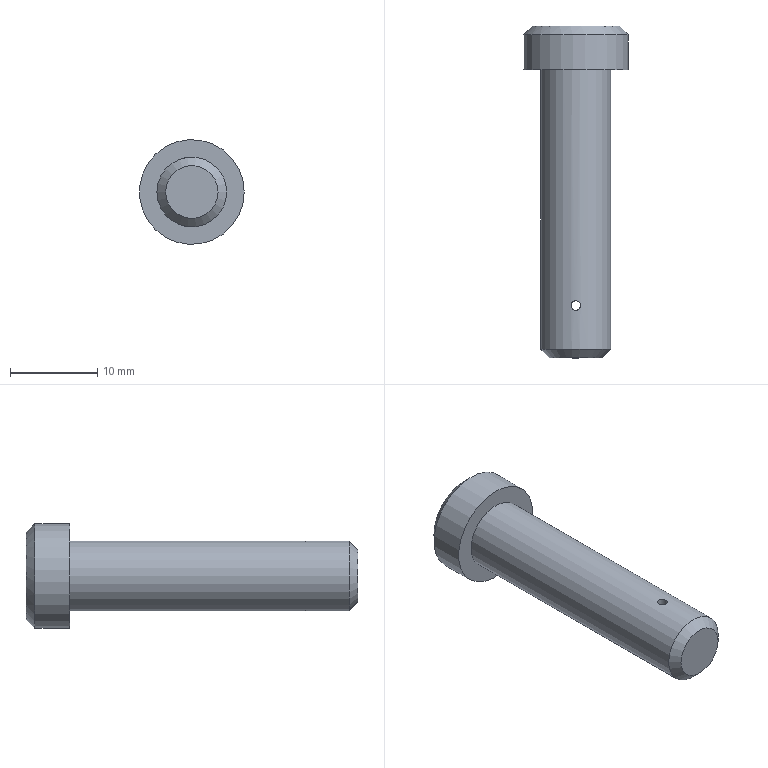Component | NX | SHAFT | 1 solid | 8 faces | box 12 x 38 x 12 mm | volume 2187 mm3 | cylinder 3 | plane 3 | cone 2 | commonest cylinder face diameters 8 x1 12 x1 1.1 x1
STEP:
#1=CARTESIAN_POINT('',(0.,0.,0.));
#2=DIRECTION('',(0.,0.,1.));
#3=DIRECTION('',(1.,0.,0.));
#4=AXIS2_PLACEMENT_3D('',#1,#2,#3);
#5=CARTESIAN_POINT('',(-77.,-19.5,-1.));
#6=VERTEX_POINT('',#5);
#7=CARTESIAN_POINT('',(-69.,-19.5,-1.));
#8=VERTEX_POINT('',#7);
#9=CARTESIAN_POINT('',(-73.,-19.5,-1.));
#10=DIRECTION('',(0.,1.,0.));
#11=DIRECTION('',(-1.,0.,0.));
#12=AXIS2_PLACEMENT_3D('',#9,#10,#11);
#13=CIRCLE('',#12,4.);
#14=CARTESIAN_POINT('',(-73.,-20.5,-1.));
#15=DIRECTION('',(0.,1.,0.));
#16=DIRECTION('',(1.,0.,0.));
#17=AXIS2_PLACEMENT_3D('',#14,#15,#16);
#18=CYLINDRICAL_SURFACE('',#17,4.);
#19=CARTESIAN_POINT('',(3.142,1.));
#20=DIRECTION('',(1.,0.));
#21=VECTOR('',#20,1.);
#22=LINE('',#19,#21);
#23=(GEOMETRIC_REPRESENTATION_CONTEXT(2)PARAMETRIC_REPRESENTATION_CONTEXT()REPRESENTATION_CONTEXT('',''));
#24=DEFINITIONAL_REPRESENTATION('',(#22),#23);
#25=PCURVE('',#18,#24);
#26=CARTESIAN_POINT('',(-73.,-19.5,-1.));
#27=DIRECTION('',(0.,1.,0.));
#28=DIRECTION('',(1.,0.,0.));
#29=AXIS2_PLACEMENT_3D('',#26,#27,#28);
#30=CONICAL_SURFACE('',#29,4.,0.7854);
#31=CARTESIAN_POINT('',(3.142,0.));
#32=DIRECTION('',(1.,0.));
#33=VECTOR('',#32,1.);
#34=LINE('',#31,#33);
#35=(GEOMETRIC_REPRESENTATION_CONTEXT(2)PARAMETRIC_REPRESENTATION_CONTEXT()REPRESENTATION_CONTEXT('',''));
#36=DEFINITIONAL_REPRESENTATION('',(#34),#35);
#37=PCURVE('',#30,#36);
#38=SURFACE_CURVE('',#13,(#25,#37),.PCURVE_S1.);
#39=EDGE_CURVE('',#6,#8,#38,.T.);
#40=ORIENTED_EDGE('',*,*,#39,.T.);
#41=CARTESIAN_POINT('',(-69.,12.5,-1.));
#42=VERTEX_POINT('',#41);
#43=CARTESIAN_POINT('',(-69.,-19.5,-1.));
#44=CARTESIAN_POINT('',(-69.,12.5,-1.));
#45=B_SPLINE_CURVE_WITH_KNOTS('',1,(#43,#44),.UNSPECIFIED.,.F.,.F.,(2,2),(1.,33.),.PIECEWISE_BEZIER_KNOTS.);
#46=CARTESIAN_POINT('',(6.283,0.));
#47=DIRECTION('',(0.,1.));
#48=VECTOR('',#47,1.);
#49=LINE('',#46,#48);
#50=(GEOMETRIC_REPRESENTATION_CONTEXT(2)PARAMETRIC_REPRESENTATION_CONTEXT()REPRESENTATION_CONTEXT('',''));
#51=DEFINITIONAL_REPRESENTATION('',(#49),#50);
#52=PCURVE('',#18,#51);
#53=CARTESIAN_POINT('',(0.,0.));
#54=DIRECTION('',(0.,1.));
#55=VECTOR('',#54,1.);
#56=LINE('',#53,#55);
#57=(GEOMETRIC_REPRESENTATION_CONTEXT(2)PARAMETRIC_REPRESENTATION_CONTEXT()REPRESENTATION_CONTEXT('',''));
#58=DEFINITIONAL_REPRESENTATION('',(#56),#57);
#59=PCURVE('',#18,#58);
#60=SEAM_CURVE('',#45,(#52,#59),.PCURVE_S1.);
#61=EDGE_CURVE('',#8,#42,#60,.T.);
#62=ORIENTED_EDGE('',*,*,#61,.T.);
#63=CARTESIAN_POINT('',(-73.,12.5,-1.));
#64=DIRECTION('',(0.,-1.,0.));
#65=DIRECTION('',(1.,0.,0.));
#66=AXIS2_PLACEMENT_3D('',#63,#64,#65);
#67=CIRCLE('',#66,4.);
#68=CARTESIAN_POINT('',(6.283,33.));
#69=DIRECTION('',(-1.,0.));
#70=VECTOR('',#69,1.);
#71=LINE('',#68,#70);
#72=(GEOMETRIC_REPRESENTATION_CONTEXT(2)PARAMETRIC_REPRESENTATION_CONTEXT()REPRESENTATION_CONTEXT('',''));
#73=DEFINITIONAL_REPRESENTATION('',(#71),#72);
#74=PCURVE('',#18,#73);
#75=CARTESIAN_POINT('',(-73.,12.5,-1.));
#76=DIRECTION('',(0.,-1.,0.));
#77=DIRECTION('',(-1.,0.,0.));
#78=AXIS2_PLACEMENT_3D('',#75,#76,#77);
#79=PLANE('',#78);
#80=CARTESIAN_POINT('',(0.,0.));
#81=DIRECTION('',(-1.,0.));
#82=AXIS2_PLACEMENT_2D('',#80,#81);
#83=CIRCLE('',#82,4.);
#84=(GEOMETRIC_REPRESENTATION_CONTEXT(2)PARAMETRIC_REPRESENTATION_CONTEXT()REPRESENTATION_CONTEXT('',''));
#85=DEFINITIONAL_REPRESENTATION('',(#83),#84);
#86=PCURVE('',#79,#85);
#87=SURFACE_CURVE('',#67,(#74,#86),.PCURVE_S1.);
#88=EDGE_CURVE('',#42,#42,#87,.T.);
#89=ORIENTED_EDGE('',*,*,#88,.T.);
#90=ORIENTED_EDGE('',*,*,#61,.F.);
#91=CARTESIAN_POINT('',(-73.,-19.5,-1.));
#92=DIRECTION('',(0.,1.,0.));
#93=DIRECTION('',(-1.,0.,0.));
#94=AXIS2_PLACEMENT_3D('',#91,#92,#93);
#95=CIRCLE('',#94,4.);
#96=CARTESIAN_POINT('',(-3.142,1.));
#97=DIRECTION('',(1.,0.));
#98=VECTOR('',#97,1.);
#99=LINE('',#96,#98);
#100=(GEOMETRIC_REPRESENTATION_CONTEXT(2)PARAMETRIC_REPRESENTATION_CONTEXT()REPRESENTATION_CONTEXT('',''));
#101=DEFINITIONAL_REPRESENTATION('',(#99),#100);
#102=PCURVE('',#18,#101);
#103=CARTESIAN_POINT('',(3.142,0.));
#104=DIRECTION('',(1.,0.));
#105=VECTOR('',#104,1.);
#106=LINE('',#103,#105);
#107=(GEOMETRIC_REPRESENTATION_CONTEXT(2)PARAMETRIC_REPRESENTATION_CONTEXT()REPRESENTATION_CONTEXT('',''));
#108=DEFINITIONAL_REPRESENTATION('',(#106),#107);
#109=PCURVE('',#30,#108);
#110=SURFACE_CURVE('',#95,(#102,#109),.PCURVE_S1.);
#111=EDGE_CURVE('',#8,#6,#110,.T.);
#112=ORIENTED_EDGE('',*,*,#111,.T.);
#113=EDGE_LOOP('',(#40,#62,#89,#90,#112));
#114=FACE_BOUND('',#113,.T.);
#115=CARTESIAN_POINT('',(-73.,-13.95,-5.));
#116=VERTEX_POINT('',#115);
#117=CARTESIAN_POINT('',(-73.,-13.95,-5.));
#118=CARTESIAN_POINT('',(-73.061,-13.95,-5.));
#119=CARTESIAN_POINT('',(-73.123,-13.961,-4.999));
#120=CARTESIAN_POINT('',(-73.181,-13.981,-4.996));
#121=CARTESIAN_POINT('',(-73.239,-14.001,-4.993));
#122=CARTESIAN_POINT('',(-73.294,-14.031,-4.989));
#123=CARTESIAN_POINT('',(-73.342,-14.069,-4.985));
#124=CARTESIAN_POINT('',(-73.39,-14.107,-4.981));
#125=CARTESIAN_POINT('',(-73.432,-14.154,-4.977));
#126=CARTESIAN_POINT('',(-73.465,-14.206,-4.973));
#127=CARTESIAN_POINT('',(-73.498,-14.258,-4.969));
#128=CARTESIAN_POINT('',(-73.522,-14.317,-4.966));
#129=CARTESIAN_POINT('',(-73.536,-14.377,-4.964));
#130=CARTESIAN_POINT('',(-73.55,-14.437,-4.962));
#131=CARTESIAN_POINT('',(-73.553,-14.5,-4.962));
#132=CARTESIAN_POINT('',(-73.547,-14.561,-4.962));
#133=CARTESIAN_POINT('',(-73.54,-14.622,-4.963));
#134=CARTESIAN_POINT('',(-73.523,-14.682,-4.966));
#135=CARTESIAN_POINT('',(-73.496,-14.737,-4.969));
#136=CARTESIAN_POINT('',(-73.47,-14.792,-4.972));
#137=CARTESIAN_POINT('',(-73.434,-14.844,-4.977));
#138=CARTESIAN_POINT('',(-73.391,-14.887,-4.981));
#139=CARTESIAN_POINT('',(-73.347,-14.931,-4.985));
#140=CARTESIAN_POINT('',(-73.296,-14.968,-4.989));
#141=CARTESIAN_POINT('',(-73.241,-14.995,-4.993));
#142=CARTESIAN_POINT('',(-73.185,-15.022,-4.996));
#143=CARTESIAN_POINT('',(-73.124,-15.039,-4.999));
#144=CARTESIAN_POINT('',(-73.063,-15.046,-5.));
#145=CARTESIAN_POINT('',(-73.002,-15.053,-5.));
#146=CARTESIAN_POINT('',(-72.939,-15.05,-5.));
#147=CARTESIAN_POINT('',(-72.879,-15.037,-4.998));
#148=CARTESIAN_POINT('',(-72.82,-15.023,-4.996));
#149=CARTESIAN_POINT('',(-72.762,-14.999,-4.993));
#150=CARTESIAN_POINT('',(-72.71,-14.967,-4.989));
#151=CARTESIAN_POINT('',(-72.658,-14.935,-4.986));
#152=CARTESIAN_POINT('',(-72.611,-14.893,-4.981));
#153=CARTESIAN_POINT('',(-72.572,-14.846,-4.977));
#154=CARTESIAN_POINT('',(-72.534,-14.798,-4.973));
#155=CARTESIAN_POINT('',(-72.502,-14.742,-4.969));
#156=CARTESIAN_POINT('',(-72.482,-14.684,-4.966));
#157=CARTESIAN_POINT('',(-72.461,-14.626,-4.964));
#158=CARTESIAN_POINT('',(-72.45,-14.564,-4.962));
#159=CARTESIAN_POINT('',(-72.45,-14.502,-4.962));
#160=CARTESIAN_POINT('',(-72.45,-14.441,-4.962));
#161=CARTESIAN_POINT('',(-72.46,-14.379,-4.963));
#162=CARTESIAN_POINT('',(-72.48,-14.321,-4.966));
#163=CARTESIAN_POINT('',(-72.5,-14.264,-4.969));
#164=CARTESIAN_POINT('',(-72.53,-14.209,-4.972));
#165=CARTESIAN_POINT('',(-72.567,-14.161,-4.977));
#166=CARTESIAN_POINT('',(-72.605,-14.112,-4.981));
#167=CARTESIAN_POINT('',(-72.652,-14.07,-4.985));
#168=CARTESIAN_POINT('',(-72.704,-14.037,-4.989));
#169=CARTESIAN_POINT('',(-72.756,-14.003,-4.993));
#170=CARTESIAN_POINT('',(-72.814,-13.979,-4.996));
#171=CARTESIAN_POINT('',(-72.874,-13.965,-4.998));
#172=CARTESIAN_POINT('',(-72.915,-13.955,-4.999));
#173=CARTESIAN_POINT('',(-72.958,-13.95,-5.));
#174=CARTESIAN_POINT('',(-73.,-13.95,-5.));
#175=B_SPLINE_CURVE_WITH_KNOTS('',3,(#117,#118,#119,#120,#121,#122,#123,#124,#125,#126,#127,#128,#129,#130,#131,#132,#133,#134,#135,#136,#137,#138,#139,#140,#141,#142,#143,#144,#145,#146,#147,#148,#149,#150,#151,#152,#153,#154,#155,#156,#157,#158,#159,#160,#161,#162,#163,#164,#165,#166,#167,#168,#169,#170,#171,#172,#173,#174),.UNSPECIFIED.,.T.,.F.,(1,3,3,3,3,3,3,3,3,3,3,3,3,3,3,3,3,3,3,3,3,1),(-0.03651,0.,0.05336,0.1067,0.1604,0.2142,0.2678,0.3209,0.3743,0.4281,0.4819,0.5353,0.5884,0.6419,0.6958,0.7495,0.8027,0.856,0.9096,0.9635,1.,1.053),.UNSPECIFIED.);
#176=CARTESIAN_POINT('',(1.571,6.55));
#177=CARTESIAN_POINT('',(1.574,6.55));
#178=CARTESIAN_POINT('',(1.581,6.549));
#179=CARTESIAN_POINT('',(1.59,6.545));
#180=CARTESIAN_POINT('',(1.6,6.538));
#181=CARTESIAN_POINT('',(1.61,6.528));
#182=CARTESIAN_POINT('',(1.619,6.516));
#183=CARTESIAN_POINT('',(1.628,6.501));
#184=CARTESIAN_POINT('',(1.637,6.483));
#185=CARTESIAN_POINT('',(1.645,6.463));
#186=CARTESIAN_POINT('',(1.653,6.441));
#187=CARTESIAN_POINT('',(1.661,6.416));
#188=CARTESIAN_POINT('',(1.668,6.389));
#189=CARTESIAN_POINT('',(1.675,6.361));
#190=CARTESIAN_POINT('',(1.681,6.33));
#191=CARTESIAN_POINT('',(1.687,6.298));
#192=CARTESIAN_POINT('',(1.692,6.264));
#193=CARTESIAN_POINT('',(1.696,6.229));
#194=CARTESIAN_POINT('',(1.7,6.193));
#195=CARTESIAN_POINT('',(1.703,6.155));
#196=CARTESIAN_POINT('',(1.706,6.117));
#197=CARTESIAN_POINT('',(1.707,6.079));
#198=CARTESIAN_POINT('',(1.708,6.039));
#199=CARTESIAN_POINT('',(1.709,6.));
#200=CARTESIAN_POINT('',(1.708,5.961));
#201=CARTESIAN_POINT('',(1.707,5.922));
#202=CARTESIAN_POINT('',(1.706,5.883));
#203=CARTESIAN_POINT('',(1.703,5.845));
#204=CARTESIAN_POINT('',(1.7,5.808));
#205=CARTESIAN_POINT('',(1.696,5.771));
#206=CARTESIAN_POINT('',(1.692,5.736));
#207=CARTESIAN_POINT('',(1.687,5.703));
#208=CARTESIAN_POINT('',(1.681,5.67));
#209=CARTESIAN_POINT('',(1.675,5.64));
#210=CARTESIAN_POINT('',(1.668,5.611));
#211=CARTESIAN_POINT('',(1.661,5.584));
#212=CARTESIAN_POINT('',(1.653,5.56));
#213=CARTESIAN_POINT('',(1.645,5.537));
#214=CARTESIAN_POINT('',(1.637,5.517));
#215=CARTESIAN_POINT('',(1.628,5.499));
#216=CARTESIAN_POINT('',(1.619,5.484));
#217=CARTESIAN_POINT('',(1.61,5.472));
#218=CARTESIAN_POINT('',(1.6,5.462));
#219=CARTESIAN_POINT('',(1.59,5.455));
#220=CARTESIAN_POINT('',(1.581,5.451));
#221=CARTESIAN_POINT('',(1.571,5.45));
#222=CARTESIAN_POINT('',(1.561,5.451));
#223=CARTESIAN_POINT('',(1.551,5.455));
#224=CARTESIAN_POINT('',(1.542,5.462));
#225=CARTESIAN_POINT('',(1.532,5.472));
#226=CARTESIAN_POINT('',(1.523,5.484));
#227=CARTESIAN_POINT('',(1.514,5.499));
#228=CARTESIAN_POINT('',(1.505,5.517));
#229=CARTESIAN_POINT('',(1.496,5.537));
#230=CARTESIAN_POINT('',(1.488,5.559));
#231=CARTESIAN_POINT('',(1.481,5.584));
#232=CARTESIAN_POINT('',(1.473,5.611));
#233=CARTESIAN_POINT('',(1.467,5.639));
#234=CARTESIAN_POINT('',(1.46,5.67));
#235=CARTESIAN_POINT('',(1.455,5.702));
#236=CARTESIAN_POINT('',(1.45,5.736));
#237=CARTESIAN_POINT('',(1.445,5.771));
#238=CARTESIAN_POINT('',(1.442,5.807));
#239=CARTESIAN_POINT('',(1.438,5.844));
#240=CARTESIAN_POINT('',(1.436,5.882));
#241=CARTESIAN_POINT('',(1.434,5.921));
#242=CARTESIAN_POINT('',(1.433,5.96));
#243=CARTESIAN_POINT('',(1.433,5.999));
#244=CARTESIAN_POINT('',(1.433,6.039));
#245=CARTESIAN_POINT('',(1.434,6.078));
#246=CARTESIAN_POINT('',(1.436,6.117));
#247=CARTESIAN_POINT('',(1.438,6.155));
#248=CARTESIAN_POINT('',(1.441,6.192));
#249=CARTESIAN_POINT('',(1.445,6.228));
#250=CARTESIAN_POINT('',(1.45,6.263));
#251=CARTESIAN_POINT('',(1.455,6.297));
#252=CARTESIAN_POINT('',(1.46,6.33));
#253=CARTESIAN_POINT('',(1.467,6.36));
#254=CARTESIAN_POINT('',(1.473,6.389));
#255=CARTESIAN_POINT('',(1.48,6.416));
#256=CARTESIAN_POINT('',(1.488,6.44));
#257=CARTESIAN_POINT('',(1.496,6.463));
#258=CARTESIAN_POINT('',(1.505,6.483));
#259=CARTESIAN_POINT('',(1.513,6.5));
#260=CARTESIAN_POINT('',(1.523,6.515));
#261=CARTESIAN_POINT('',(1.532,6.528));
#262=CARTESIAN_POINT('',(1.541,6.538));
#263=CARTESIAN_POINT('',(1.551,6.545));
#264=CARTESIAN_POINT('',(1.561,6.549));
#265=CARTESIAN_POINT('',(1.568,6.55));
#266=CARTESIAN_POINT('',(1.571,6.55));
#267=B_SPLINE_CURVE_WITH_KNOTS('',3,(#176,#177,#178,#179,#180,#181,#182,#183,#184,#185,#186,#187,#188,#189,#190,#191,#192,#193,#194,#195,#196,#197,#198,#199,#200,#201,#202,#203,#204,#205,#206,#207,#208,#209,#210,#211,#212,#213,#214,#215,#216,#217,#218,#219,#220,#221,#222,#223,#224,#225,#226,#227,#228,#229,#230,#231,#232,#233,#234,#235,#236,#237,#238,#239,#240,#241,#242,#243,#244,#245,#246,#247,#248,#249,#250,#251,#252,#253,#254,#255,#256,#257,#258,#259,#260,#261,#262,#263,#264,#265,#266),.UNSPECIFIED.,.T.,.F.,(4,1,1,1,1,1,1,1,1,1,1,1,1,1,1,1,1,1,1,1,1,1,1,1,1,1,1,1,1,1,1,1,1,1,1,1,1,1,1,1,1,1,1,1,1,1,1,1,1,1,1,1,1,1,1,1,1,1,1,1,1,1,1,1,1,1,1,1,1,1,1,1,1,1,1,1,1,1,1,1,1,1,1,1,1,1,1,1,4),(0.,0.01136,0.02273,0.03409,0.04545,0.05682,0.06818,0.07955,0.09091,0.1023,0.1136,0.125,0.1364,0.1477,0.1591,0.1705,0.1818,0.1932,0.2045,0.2159,0.2273,0.2386,0.25,0.2614,0.2727,0.2841,0.2955,0.3068,0.3182,0.3295,0.3409,0.3523,0.3636,0.375,0.3864,0.3977,0.4091,0.4205,0.4318,0.4432,0.4545,0.4659,0.4773,0.4886,0.5,0.5114,0.5227,0.5341,0.5455,0.5568,0.5682,0.5795,0.5909,0.6023,0.6136,0.625,0.6364,0.6477,0.6591,0.6705,0.6818,0.6932,0.7045,0.7159,0.7273,0.7386,0.75,0.7614,0.7727,0.7841,0.7955,0.8068,0.8182,0.8295,0.8409,0.8523,0.8636,0.875,0.8864,0.8977,0.9091,0.9205,0.9318,0.9432,0.9545,0.9659,0.9773,0.9886,1.),.QUASI_UNIFORM_KNOTS.);
#268=(GEOMETRIC_REPRESENTATION_CONTEXT(2)PARAMETRIC_REPRESENTATION_CONTEXT()REPRESENTATION_CONTEXT('',''));
#269=DEFINITIONAL_REPRESENTATION('',(#267),#268);
#270=PCURVE('',#18,#269);
#271=CARTESIAN_POINT('',(-73.,-14.5,29.));
#272=DIRECTION('',(0.,0.,-1.));
#273=DIRECTION('',(0.,1.,0.));
#274=AXIS2_PLACEMENT_3D('',#271,#272,#273);
#275=CYLINDRICAL_SURFACE('',#274,0.55);
#276=CARTESIAN_POINT('',(6.283,34.));
#277=CARTESIAN_POINT('',(0.,34.));
#278=B_SPLINE_CURVE_WITH_KNOTS('',1,(#276,#277),.UNSPECIFIED.,.F.,.F.,(2,2),(0.,1.),.PIECEWISE_BEZIER_KNOTS.);
#279=(GEOMETRIC_REPRESENTATION_CONTEXT(2)PARAMETRIC_REPRESENTATION_CONTEXT()REPRESENTATION_CONTEXT('',''));
#280=DEFINITIONAL_REPRESENTATION('',(#278),#279);
#281=PCURVE('',#275,#280);
#282=SURFACE_CURVE('',#175,(#270,#281),.PCURVE_S1.);
#283=EDGE_CURVE('',#116,#116,#282,.T.);
#284=ORIENTED_EDGE('',*,*,#283,.T.);
#285=EDGE_LOOP('',(#284));
#286=FACE_BOUND('',#285,.T.);
#287=CARTESIAN_POINT('',(-73.,-13.95,3.));
#288=VERTEX_POINT('',#287);
#289=CARTESIAN_POINT('',(-73.,-13.95,3.));
#290=CARTESIAN_POINT('',(-72.939,-13.95,3.));
#291=CARTESIAN_POINT('',(-72.877,-13.961,2.999));
#292=CARTESIAN_POINT('',(-72.819,-13.981,2.996));
#293=CARTESIAN_POINT('',(-72.761,-14.001,2.993));
#294=CARTESIAN_POINT('',(-72.706,-14.031,2.989));
#295=CARTESIAN_POINT('',(-72.658,-14.069,2.985));
#296=CARTESIAN_POINT('',(-72.61,-14.107,2.981));
#297=CARTESIAN_POINT('',(-72.568,-14.154,2.977));
#298=CARTESIAN_POINT('',(-72.535,-14.206,2.973));
#299=CARTESIAN_POINT('',(-72.502,-14.258,2.969));
#300=CARTESIAN_POINT('',(-72.478,-14.317,2.966));
#301=CARTESIAN_POINT('',(-72.464,-14.377,2.964));
#302=CARTESIAN_POINT('',(-72.45,-14.437,2.962));
#303=CARTESIAN_POINT('',(-72.447,-14.5,2.962));
#304=CARTESIAN_POINT('',(-72.453,-14.561,2.962));
#305=CARTESIAN_POINT('',(-72.46,-14.622,2.963));
#306=CARTESIAN_POINT('',(-72.477,-14.682,2.966));
#307=CARTESIAN_POINT('',(-72.504,-14.737,2.969));
#308=CARTESIAN_POINT('',(-72.53,-14.792,2.972));
#309=CARTESIAN_POINT('',(-72.566,-14.844,2.977));
#310=CARTESIAN_POINT('',(-72.609,-14.887,2.981));
#311=CARTESIAN_POINT('',(-72.653,-14.931,2.985));
#312=CARTESIAN_POINT('',(-72.704,-14.968,2.989));
#313=CARTESIAN_POINT('',(-72.759,-14.995,2.993));
#314=CARTESIAN_POINT('',(-72.815,-15.022,2.996));
#315=CARTESIAN_POINT('',(-72.876,-15.039,2.999));
#316=CARTESIAN_POINT('',(-72.937,-15.046,3.));
#317=CARTESIAN_POINT('',(-72.998,-15.053,3.));
#318=CARTESIAN_POINT('',(-73.061,-15.05,3.));
#319=CARTESIAN_POINT('',(-73.121,-15.037,2.998));
#320=CARTESIAN_POINT('',(-73.18,-15.023,2.996));
#321=CARTESIAN_POINT('',(-73.238,-14.999,2.993));
#322=CARTESIAN_POINT('',(-73.29,-14.967,2.989));
#323=CARTESIAN_POINT('',(-73.342,-14.935,2.986));
#324=CARTESIAN_POINT('',(-73.389,-14.893,2.981));
#325=CARTESIAN_POINT('',(-73.428,-14.846,2.977));
#326=CARTESIAN_POINT('',(-73.466,-14.798,2.973));
#327=CARTESIAN_POINT('',(-73.498,-14.742,2.969));
#328=CARTESIAN_POINT('',(-73.518,-14.684,2.966));
#329=CARTESIAN_POINT('',(-73.539,-14.626,2.964));
#330=CARTESIAN_POINT('',(-73.55,-14.564,2.962));
#331=CARTESIAN_POINT('',(-73.55,-14.502,2.962));
#332=CARTESIAN_POINT('',(-73.55,-14.441,2.962));
#333=CARTESIAN_POINT('',(-73.54,-14.379,2.963));
#334=CARTESIAN_POINT('',(-73.52,-14.321,2.966));
#335=CARTESIAN_POINT('',(-73.5,-14.264,2.969));
#336=CARTESIAN_POINT('',(-73.47,-14.209,2.972));
#337=CARTESIAN_POINT('',(-73.433,-14.161,2.977));
#338=CARTESIAN_POINT('',(-73.395,-14.112,2.981));
#339=CARTESIAN_POINT('',(-73.348,-14.07,2.985));
#340=CARTESIAN_POINT('',(-73.296,-14.037,2.989));
#341=CARTESIAN_POINT('',(-73.244,-14.003,2.993));
#342=CARTESIAN_POINT('',(-73.186,-13.979,2.996));
#343=CARTESIAN_POINT('',(-73.126,-13.965,2.998));
#344=CARTESIAN_POINT('',(-73.085,-13.955,2.999));
#345=CARTESIAN_POINT('',(-73.042,-13.95,3.));
#346=CARTESIAN_POINT('',(-73.,-13.95,3.));
#347=B_SPLINE_CURVE_WITH_KNOTS('',3,(#289,#290,#291,#292,#293,#294,#295,#296,#297,#298,#299,#300,#301,#302,#303,#304,#305,#306,#307,#308,#309,#310,#311,#312,#313,#314,#315,#316,#317,#318,#319,#320,#321,#322,#323,#324,#325,#326,#327,#328,#329,#330,#331,#332,#333,#334,#335,#336,#337,#338,#339,#340,#341,#342,#343,#344,#345,#346),.UNSPECIFIED.,.T.,.F.,(1,3,3,3,3,3,3,3,3,3,3,3,3,3,3,3,3,3,3,3,3,1),(-0.03651,0.,0.05336,0.1067,0.1604,0.2142,0.2678,0.3209,0.3743,0.4281,0.4819,0.5353,0.5884,0.6419,0.6958,0.7495,0.8027,0.856,0.9096,0.9635,1.,1.053),.UNSPECIFIED.);
#348=CARTESIAN_POINT('',(4.712,6.55));
#349=CARTESIAN_POINT('',(4.716,6.55));
#350=CARTESIAN_POINT('',(4.722,6.549));
#351=CARTESIAN_POINT('',(4.732,6.545));
#352=CARTESIAN_POINT('',(4.742,6.538));
#353=CARTESIAN_POINT('',(4.751,6.528));
#354=CARTESIAN_POINT('',(4.761,6.516));
#355=CARTESIAN_POINT('',(4.77,6.501));
#356=CARTESIAN_POINT('',(4.778,6.483));
#357=CARTESIAN_POINT('',(4.787,6.463));
#358=CARTESIAN_POINT('',(4.795,6.441));
#359=CARTESIAN_POINT('',(4.803,6.416));
#360=CARTESIAN_POINT('',(4.81,6.389));
#361=CARTESIAN_POINT('',(4.817,6.361));
#362=CARTESIAN_POINT('',(4.823,6.33));
#363=CARTESIAN_POINT('',(4.828,6.298));
#364=CARTESIAN_POINT('',(4.833,6.264));
#365=CARTESIAN_POINT('',(4.838,6.229));
#366=CARTESIAN_POINT('',(4.842,6.193));
#367=CARTESIAN_POINT('',(4.845,6.155));
#368=CARTESIAN_POINT('',(4.847,6.117));
#369=CARTESIAN_POINT('',(4.849,6.079));
#370=CARTESIAN_POINT('',(4.85,6.039));
#371=CARTESIAN_POINT('',(4.85,6.));
#372=CARTESIAN_POINT('',(4.85,5.961));
#373=CARTESIAN_POINT('',(4.849,5.922));
#374=CARTESIAN_POINT('',(4.847,5.883));
#375=CARTESIAN_POINT('',(4.845,5.845));
#376=CARTESIAN_POINT('',(4.842,5.808));
#377=CARTESIAN_POINT('',(4.838,5.771));
#378=CARTESIAN_POINT('',(4.833,5.736));
#379=CARTESIAN_POINT('',(4.828,5.703));
#380=CARTESIAN_POINT('',(4.823,5.67));
#381=CARTESIAN_POINT('',(4.817,5.64));
#382=CARTESIAN_POINT('',(4.81,5.611));
#383=CARTESIAN_POINT('',(4.803,5.584));
#384=CARTESIAN_POINT('',(4.795,5.56));
#385=CARTESIAN_POINT('',(4.787,5.537));
#386=CARTESIAN_POINT('',(4.778,5.517));
#387=CARTESIAN_POINT('',(4.77,5.499));
#388=CARTESIAN_POINT('',(4.761,5.484));
#389=CARTESIAN_POINT('',(4.751,5.472));
#390=CARTESIAN_POINT('',(4.742,5.462));
#391=CARTESIAN_POINT('',(4.732,5.455));
#392=CARTESIAN_POINT('',(4.722,5.451));
#393=CARTESIAN_POINT('',(4.712,5.45));
#394=CARTESIAN_POINT('',(4.703,5.451));
#395=CARTESIAN_POINT('',(4.693,5.455));
#396=CARTESIAN_POINT('',(4.683,5.462));
#397=CARTESIAN_POINT('',(4.674,5.472));
#398=CARTESIAN_POINT('',(4.664,5.484));
#399=CARTESIAN_POINT('',(4.655,5.499));
#400=CARTESIAN_POINT('',(4.646,5.517));
#401=CARTESIAN_POINT('',(4.638,5.537));
#402=CARTESIAN_POINT('',(4.63,5.559));
#403=CARTESIAN_POINT('',(4.622,5.584));
#404=CARTESIAN_POINT('',(4.615,5.611));
#405=CARTESIAN_POINT('',(4.608,5.639));
#406=CARTESIAN_POINT('',(4.602,5.67));
#407=CARTESIAN_POINT('',(4.596,5.702));
#408=CARTESIAN_POINT('',(4.591,5.736));
#409=CARTESIAN_POINT('',(4.587,5.771));
#410=CARTESIAN_POINT('',(4.583,5.807));
#411=CARTESIAN_POINT('',(4.58,5.844));
#412=CARTESIAN_POINT('',(4.578,5.882));
#413=CARTESIAN_POINT('',(4.576,5.921));
#414=CARTESIAN_POINT('',(4.575,5.96));
#415=CARTESIAN_POINT('',(4.574,5.999));
#416=CARTESIAN_POINT('',(4.575,6.039));
#417=CARTESIAN_POINT('',(4.576,6.078));
#418=CARTESIAN_POINT('',(4.578,6.117));
#419=CARTESIAN_POINT('',(4.58,6.155));
#420=CARTESIAN_POINT('',(4.583,6.192));
#421=CARTESIAN_POINT('',(4.587,6.228));
#422=CARTESIAN_POINT('',(4.591,6.263));
#423=CARTESIAN_POINT('',(4.596,6.297));
#424=CARTESIAN_POINT('',(4.602,6.33));
#425=CARTESIAN_POINT('',(4.608,6.36));
#426=CARTESIAN_POINT('',(4.615,6.389));
#427=CARTESIAN_POINT('',(4.622,6.416));
#428=CARTESIAN_POINT('',(4.63,6.44));
#429=CARTESIAN_POINT('',(4.638,6.463));
#430=CARTESIAN_POINT('',(4.646,6.483));
#431=CARTESIAN_POINT('',(4.655,6.5));
#432=CARTESIAN_POINT('',(4.664,6.515));
#433=CARTESIAN_POINT('',(4.673,6.528));
#434=CARTESIAN_POINT('',(4.683,6.538));
#435=CARTESIAN_POINT('',(4.693,6.545));
#436=CARTESIAN_POINT('',(4.703,6.549));
#437=CARTESIAN_POINT('',(4.709,6.55));
#438=CARTESIAN_POINT('',(4.712,6.55));
#439=B_SPLINE_CURVE_WITH_KNOTS('',3,(#348,#349,#350,#351,#352,#353,#354,#355,#356,#357,#358,#359,#360,#361,#362,#363,#364,#365,#366,#367,#368,#369,#370,#371,#372,#373,#374,#375,#376,#377,#378,#379,#380,#381,#382,#383,#384,#385,#386,#387,#388,#389,#390,#391,#392,#393,#394,#395,#396,#397,#398,#399,#400,#401,#402,#403,#404,#405,#406,#407,#408,#409,#410,#411,#412,#413,#414,#415,#416,#417,#418,#419,#420,#421,#422,#423,#424,#425,#426,#427,#428,#429,#430,#431,#432,#433,#434,#435,#436,#437,#438),.UNSPECIFIED.,.T.,.F.,(4,1,1,1,1,1,1,1,1,1,1,1,1,1,1,1,1,1,1,1,1,1,1,1,1,1,1,1,1,1,1,1,1,1,1,1,1,1,1,1,1,1,1,1,1,1,1,1,1,1,1,1,1,1,1,1,1,1,1,1,1,1,1,1,1,1,1,1,1,1,1,1,1,1,1,1,1,1,1,1,1,1,1,1,1,1,1,1,4),(0.,0.01136,0.02273,0.03409,0.04545,0.05682,0.06818,0.07955,0.09091,0.1023,0.1136,0.125,0.1364,0.1477,0.1591,0.1705,0.1818,0.1932,0.2045,0.2159,0.2273,0.2386,0.25,0.2614,0.2727,0.2841,0.2955,0.3068,0.3182,0.3295,0.3409,0.3523,0.3636,0.375,0.3864,0.3977,0.4091,0.4205,0.4318,0.4432,0.4545,0.4659,0.4773,0.4886,0.5,0.5114,0.5227,0.5341,0.5455,0.5568,0.5682,0.5795,0.5909,0.6023,0.6136,0.625,0.6364,0.6477,0.6591,0.6705,0.6818,0.6932,0.7045,0.7159,0.7273,0.7386,0.75,0.7614,0.7727,0.7841,0.7955,0.8068,0.8182,0.8295,0.8409,0.8523,0.8636,0.875,0.8864,0.8977,0.9091,0.9205,0.9318,0.9432,0.9545,0.9659,0.9773,0.9886,1.),.QUASI_UNIFORM_KNOTS.);
#440=(GEOMETRIC_REPRESENTATION_CONTEXT(2)PARAMETRIC_REPRESENTATION_CONTEXT()REPRESENTATION_CONTEXT('',''));
#441=DEFINITIONAL_REPRESENTATION('',(#439),#440);
#442=PCURVE('',#18,#441);
#443=CARTESIAN_POINT('',(0.,26.));
#444=CARTESIAN_POINT('',(6.283,26.));
#445=B_SPLINE_CURVE_WITH_KNOTS('',1,(#443,#444),.UNSPECIFIED.,.F.,.F.,(2,2),(0.,1.),.PIECEWISE_BEZIER_KNOTS.);
#446=(GEOMETRIC_REPRESENTATION_CONTEXT(2)PARAMETRIC_REPRESENTATION_CONTEXT()REPRESENTATION_CONTEXT('',''));
#447=DEFINITIONAL_REPRESENTATION('',(#445),#446);
#448=PCURVE('',#275,#447);
#449=SURFACE_CURVE('',#347,(#442,#448),.PCURVE_S1.);
#450=EDGE_CURVE('',#288,#288,#449,.T.);
#451=ORIENTED_EDGE('',*,*,#450,.T.);
#452=EDGE_LOOP('',(#451));
#453=FACE_BOUND('',#452,.T.);
#454=ADVANCED_FACE('',(#114,#286,#453),#18,.T.);
#455=CARTESIAN_POINT('',(-76.,-20.5,-1.));
#456=VERTEX_POINT('',#455);
#457=CARTESIAN_POINT('',(-73.,-20.5,-1.));
#458=DIRECTION('',(0.,-1.,0.));
#459=DIRECTION('',(-1.,0.,0.));
#460=AXIS2_PLACEMENT_3D('',#457,#458,#459);
#461=CIRCLE('',#460,3.);
#462=CARTESIAN_POINT('',(-73.,-20.5,-1.));
#463=DIRECTION('',(0.,-1.,0.));
#464=DIRECTION('',(-1.,0.,0.));
#465=AXIS2_PLACEMENT_3D('',#462,#463,#464);
#466=PLANE('',#465);
#467=CARTESIAN_POINT('',(0.,0.));
#468=DIRECTION('',(1.,0.));
#469=AXIS2_PLACEMENT_2D('',#467,#468);
#470=CIRCLE('',#469,3.);
#471=(GEOMETRIC_REPRESENTATION_CONTEXT(2)PARAMETRIC_REPRESENTATION_CONTEXT()REPRESENTATION_CONTEXT('',''));
#472=DEFINITIONAL_REPRESENTATION('',(#470),#471);
#473=PCURVE('',#466,#472);
#474=CARTESIAN_POINT('',(9.425,-1.));
#475=DIRECTION('',(-1.,0.));
#476=VECTOR('',#475,1.);
#477=LINE('',#474,#476);
#478=(GEOMETRIC_REPRESENTATION_CONTEXT(2)PARAMETRIC_REPRESENTATION_CONTEXT()REPRESENTATION_CONTEXT('',''));
#479=DEFINITIONAL_REPRESENTATION('',(#477),#478);
#480=PCURVE('',#30,#479);
#481=SURFACE_CURVE('',#461,(#473,#480),.PCURVE_S1.);
#482=EDGE_CURVE('',#456,#456,#481,.T.);
#483=ORIENTED_EDGE('',*,*,#482,.T.);
#484=EDGE_LOOP('',(#483));
#485=FACE_BOUND('',#484,.T.);
#486=ADVANCED_FACE('',(#485),#466,.T.);
#487=CARTESIAN_POINT('',(-68.,17.5,-1.));
#488=VERTEX_POINT('',#487);
#489=CARTESIAN_POINT('',(-73.,17.5,-1.));
#490=DIRECTION('',(0.,1.,0.));
#491=DIRECTION('',(1.,0.,0.));
#492=AXIS2_PLACEMENT_3D('',#489,#490,#491);
#493=CIRCLE('',#492,5.);
#494=CARTESIAN_POINT('',(-73.,17.5,-1.));
#495=DIRECTION('',(0.,1.,0.));
#496=DIRECTION('',(1.,0.,0.));
#497=AXIS2_PLACEMENT_3D('',#494,#495,#496);
#498=PLANE('',#497);
#499=CARTESIAN_POINT('',(0.,0.));
#500=DIRECTION('',(1.,0.));
#501=AXIS2_PLACEMENT_2D('',#499,#500);
#502=CIRCLE('',#501,5.);
#503=(GEOMETRIC_REPRESENTATION_CONTEXT(2)PARAMETRIC_REPRESENTATION_CONTEXT()REPRESENTATION_CONTEXT('',''));
#504=DEFINITIONAL_REPRESENTATION('',(#502),#503);
#505=PCURVE('',#498,#504);
#506=CARTESIAN_POINT('',(-73.,17.5,-1.));
#507=DIRECTION('',(0.,-1.,0.));
#508=DIRECTION('',(-1.,0.,0.));
#509=AXIS2_PLACEMENT_3D('',#506,#507,#508);
#510=CONICAL_SURFACE('',#509,5.,0.7854);
#511=CARTESIAN_POINT('',(9.425,0.));
#512=DIRECTION('',(-1.,0.));
#513=VECTOR('',#512,1.);
#514=LINE('',#511,#513);
#515=(GEOMETRIC_REPRESENTATION_CONTEXT(2)PARAMETRIC_REPRESENTATION_CONTEXT()REPRESENTATION_CONTEXT('',''));
#516=DEFINITIONAL_REPRESENTATION('',(#514),#515);
#517=PCURVE('',#510,#516);
#518=SURFACE_CURVE('',#493,(#505,#517),.PCURVE_S1.);
#519=EDGE_CURVE('',#488,#488,#518,.T.);
#520=ORIENTED_EDGE('',*,*,#519,.T.);
#521=EDGE_LOOP('',(#520));
#522=FACE_BOUND('',#521,.T.);
#523=ADVANCED_FACE('',(#522),#498,.T.);
#524=ORIENTED_EDGE('',*,*,#88,.F.);
#525=EDGE_LOOP('',(#524));
#526=FACE_BOUND('',#525,.T.);
#527=CARTESIAN_POINT('',(-67.,12.5,-1.));
#528=VERTEX_POINT('',#527);
#529=CARTESIAN_POINT('',(-73.,12.5,-1.));
#530=DIRECTION('',(0.,1.,0.));
#531=DIRECTION('',(1.,0.,0.));
#532=AXIS2_PLACEMENT_3D('',#529,#530,#531);
#533=CIRCLE('',#532,6.);
#534=CARTESIAN_POINT('',(-6.,0.));
#535=CARTESIAN_POINT('',(-6.,10.392));
#536=CARTESIAN_POINT('',(3.,5.196));
#537=CARTESIAN_POINT('',(12.,0.));
#538=CARTESIAN_POINT('',(3.,-5.196));
#539=CARTESIAN_POINT('',(-6.,-10.392));
#540=CARTESIAN_POINT('',(-6.,0.));
#541=(BOUNDED_CURVE()B_SPLINE_CURVE(2,(#534,#535,#536,#537,#538,#539,#540),.UNSPECIFIED.,.T.,.F.)B_SPLINE_CURVE_WITH_KNOTS((1,2,2,2,2,1),(-2.094,0.,2.094,4.189,6.283,8.378),.UNSPECIFIED.)CURVE()GEOMETRIC_REPRESENTATION_ITEM()RATIONAL_B_SPLINE_CURVE((1.,0.5,1.,0.5,1.,0.5,1.))REPRESENTATION_ITEM(''));
#542=(GEOMETRIC_REPRESENTATION_CONTEXT(2)PARAMETRIC_REPRESENTATION_CONTEXT()REPRESENTATION_CONTEXT('',''));
#543=DEFINITIONAL_REPRESENTATION('',(#541),#542);
#544=PCURVE('',#79,#543);
#545=CARTESIAN_POINT('',(-73.,12.5,-1.));
#546=DIRECTION('',(0.,1.,0.));
#547=DIRECTION('',(1.,0.,0.));
#548=AXIS2_PLACEMENT_3D('',#545,#546,#547);
#549=CYLINDRICAL_SURFACE('',#548,6.);
#550=CARTESIAN_POINT('',(0.,0.));
#551=DIRECTION('',(1.,0.));
#552=VECTOR('',#551,1.);
#553=LINE('',#550,#552);
#554=(GEOMETRIC_REPRESENTATION_CONTEXT(2)PARAMETRIC_REPRESENTATION_CONTEXT()REPRESENTATION_CONTEXT('',''));
#555=DEFINITIONAL_REPRESENTATION('',(#553),#554);
#556=PCURVE('',#549,#555);
#557=SURFACE_CURVE('',#533,(#544,#556),.PCURVE_S1.);
#558=EDGE_CURVE('',#528,#528,#557,.T.);
#559=ORIENTED_EDGE('',*,*,#558,.F.);
#560=EDGE_LOOP('',(#559));
#561=FACE_BOUND('',#560,.T.);
#562=ADVANCED_FACE('',(#526,#561),#79,.T.);
#563=CARTESIAN_POINT('',(-67.,16.5,-1.));
#564=VERTEX_POINT('',#563);
#565=CARTESIAN_POINT('',(-73.,16.5,-1.));
#566=DIRECTION('',(0.,-1.,0.));
#567=DIRECTION('',(1.,0.,0.));
#568=AXIS2_PLACEMENT_3D('',#565,#566,#567);
#569=CIRCLE('',#568,6.);
#570=CARTESIAN_POINT('',(6.283,4.));
#571=DIRECTION('',(-1.,0.));
#572=VECTOR('',#571,1.);
#573=LINE('',#570,#572);
#574=(GEOMETRIC_REPRESENTATION_CONTEXT(2)PARAMETRIC_REPRESENTATION_CONTEXT()REPRESENTATION_CONTEXT('',''));
#575=DEFINITIONAL_REPRESENTATION('',(#573),#574);
#576=PCURVE('',#549,#575);
#577=CARTESIAN_POINT('',(3.142,1.));
#578=DIRECTION('',(1.,0.));
#579=VECTOR('',#578,1.);
#580=LINE('',#577,#579);
#581=(GEOMETRIC_REPRESENTATION_CONTEXT(2)PARAMETRIC_REPRESENTATION_CONTEXT()REPRESENTATION_CONTEXT('',''));
#582=DEFINITIONAL_REPRESENTATION('',(#580),#581);
#583=PCURVE('',#510,#582);
#584=SURFACE_CURVE('',#569,(#576,#583),.PCURVE_S1.);
#585=EDGE_CURVE('',#564,#564,#584,.T.);
#586=ORIENTED_EDGE('',*,*,#585,.T.);
#587=CARTESIAN_POINT('',(-67.,12.5,-1.));
#588=CARTESIAN_POINT('',(-67.,16.5,-1.));
#589=B_SPLINE_CURVE_WITH_KNOTS('',1,(#587,#588),.UNSPECIFIED.,.F.,.F.,(2,2),(0.,4.),.PIECEWISE_BEZIER_KNOTS.);
#590=CARTESIAN_POINT('',(0.,0.));
#591=DIRECTION('',(0.,1.));
#592=VECTOR('',#591,1.);
#593=LINE('',#590,#592);
#594=(GEOMETRIC_REPRESENTATION_CONTEXT(2)PARAMETRIC_REPRESENTATION_CONTEXT()REPRESENTATION_CONTEXT('',''));
#595=DEFINITIONAL_REPRESENTATION('',(#593),#594);
#596=PCURVE('',#549,#595);
#597=CARTESIAN_POINT('',(6.283,0.));
#598=DIRECTION('',(0.,1.));
#599=VECTOR('',#598,1.);
#600=LINE('',#597,#599);
#601=(GEOMETRIC_REPRESENTATION_CONTEXT(2)PARAMETRIC_REPRESENTATION_CONTEXT()REPRESENTATION_CONTEXT('',''));
#602=DEFINITIONAL_REPRESENTATION('',(#600),#601);
#603=PCURVE('',#549,#602);
#604=SEAM_CURVE('',#589,(#596,#603),.PCURVE_S1.);
#605=EDGE_CURVE('',#528,#564,#604,.T.);
#606=ORIENTED_EDGE('',*,*,#605,.F.);
#607=ORIENTED_EDGE('',*,*,#558,.T.);
#608=ORIENTED_EDGE('',*,*,#605,.T.);
#609=EDGE_LOOP('',(#586,#606,#607,#608));
#610=FACE_BOUND('',#609,.T.);
#611=ADVANCED_FACE('',(#610),#549,.T.);
#612=ORIENTED_EDGE('',*,*,#585,.F.);
#613=CARTESIAN_POINT('',(-68.,17.5,-1.));
#614=CARTESIAN_POINT('',(-67.,16.5,-1.));
#615=B_SPLINE_CURVE_WITH_KNOTS('',1,(#613,#614),.UNSPECIFIED.,.F.,.F.,(2,2),(0.,1.414),.PIECEWISE_BEZIER_KNOTS.);
#616=CARTESIAN_POINT('',(3.142,0.));
#617=DIRECTION('',(0.,1.));
#618=VECTOR('',#617,1.);
#619=LINE('',#616,#618);
#620=(GEOMETRIC_REPRESENTATION_CONTEXT(2)PARAMETRIC_REPRESENTATION_CONTEXT()REPRESENTATION_CONTEXT('',''));
#621=DEFINITIONAL_REPRESENTATION('',(#619),#620);
#622=PCURVE('',#510,#621);
#623=CARTESIAN_POINT('',(9.425,0.));
#624=DIRECTION('',(0.,1.));
#625=VECTOR('',#624,1.);
#626=LINE('',#623,#625);
#627=(GEOMETRIC_REPRESENTATION_CONTEXT(2)PARAMETRIC_REPRESENTATION_CONTEXT()REPRESENTATION_CONTEXT('',''));
#628=DEFINITIONAL_REPRESENTATION('',(#626),#627);
#629=PCURVE('',#510,#628);
#630=SEAM_CURVE('',#615,(#622,#629),.PCURVE_S1.);
#631=EDGE_CURVE('',#488,#564,#630,.T.);
#632=ORIENTED_EDGE('',*,*,#631,.F.);
#633=ORIENTED_EDGE('',*,*,#519,.F.);
#634=ORIENTED_EDGE('',*,*,#631,.T.);
#635=EDGE_LOOP('',(#612,#632,#633,#634));
#636=FACE_BOUND('',#635,.T.);
#637=ADVANCED_FACE('',(#636),#510,.T.);
#638=ORIENTED_EDGE('',*,*,#482,.F.);
#639=CARTESIAN_POINT('',(-76.,-20.5,-1.));
#640=CARTESIAN_POINT('',(-77.,-19.5,-1.));
#641=B_SPLINE_CURVE_WITH_KNOTS('',1,(#639,#640),.UNSPECIFIED.,.F.,.F.,(2,2),(-1.414,0.),.PIECEWISE_BEZIER_KNOTS.);
#642=CARTESIAN_POINT('',(9.425,0.));
#643=DIRECTION('',(0.,1.));
#644=VECTOR('',#643,1.);
#645=LINE('',#642,#644);
#646=(GEOMETRIC_REPRESENTATION_CONTEXT(2)PARAMETRIC_REPRESENTATION_CONTEXT()REPRESENTATION_CONTEXT('',''));
#647=DEFINITIONAL_REPRESENTATION('',(#645),#646);
#648=PCURVE('',#30,#647);
#649=CARTESIAN_POINT('',(3.142,0.));
#650=DIRECTION('',(0.,1.));
#651=VECTOR('',#650,1.);
#652=LINE('',#649,#651);
#653=(GEOMETRIC_REPRESENTATION_CONTEXT(2)PARAMETRIC_REPRESENTATION_CONTEXT()REPRESENTATION_CONTEXT('',''));
#654=DEFINITIONAL_REPRESENTATION('',(#652),#653);
#655=PCURVE('',#30,#654);
#656=SEAM_CURVE('',#641,(#648,#655),.PCURVE_S1.);
#657=EDGE_CURVE('',#456,#6,#656,.T.);
#658=ORIENTED_EDGE('',*,*,#657,.T.);
#659=ORIENTED_EDGE('',*,*,#111,.F.);
#660=ORIENTED_EDGE('',*,*,#39,.F.);
#661=ORIENTED_EDGE('',*,*,#657,.F.);
#662=EDGE_LOOP('',(#638,#658,#659,#660,#661));
#663=FACE_BOUND('',#662,.T.);
#664=ADVANCED_FACE('',(#663),#30,.T.);
#665=ORIENTED_EDGE('',*,*,#450,.T.);
#666=CARTESIAN_POINT('',(-73.,-13.95,3.));
#667=CARTESIAN_POINT('',(-73.,-13.95,-5.));
#668=B_SPLINE_CURVE_WITH_KNOTS('',1,(#666,#667),.UNSPECIFIED.,.F.,.F.,(2,2),(26.,34.),.PIECEWISE_BEZIER_KNOTS.);
#669=CARTESIAN_POINT('',(6.283,0.));
#670=DIRECTION('',(0.,1.));
#671=VECTOR('',#670,1.);
#672=LINE('',#669,#671);
#673=(GEOMETRIC_REPRESENTATION_CONTEXT(2)PARAMETRIC_REPRESENTATION_CONTEXT()REPRESENTATION_CONTEXT('',''));
#674=DEFINITIONAL_REPRESENTATION('',(#672),#673);
#675=PCURVE('',#275,#674);
#676=CARTESIAN_POINT('',(0.,0.));
#677=DIRECTION('',(0.,1.));
#678=VECTOR('',#677,1.);
#679=LINE('',#676,#678);
#680=(GEOMETRIC_REPRESENTATION_CONTEXT(2)PARAMETRIC_REPRESENTATION_CONTEXT()REPRESENTATION_CONTEXT('',''));
#681=DEFINITIONAL_REPRESENTATION('',(#679),#680);
#682=PCURVE('',#275,#681);
#683=SEAM_CURVE('',#668,(#675,#682),.PCURVE_S1.);
#684=EDGE_CURVE('',#288,#116,#683,.T.);
#685=ORIENTED_EDGE('',*,*,#684,.T.);
#686=ORIENTED_EDGE('',*,*,#283,.T.);
#687=ORIENTED_EDGE('',*,*,#684,.F.);
#688=EDGE_LOOP('',(#665,#685,#686,#687));
#689=FACE_BOUND('',#688,.F.);
#690=ADVANCED_FACE('',(#689),#275,.F.);
#691=CLOSED_SHELL('',(#454,#486,#523,#562,#611,#637,#664,#690));
#692=MANIFOLD_SOLID_BREP('',#691);
#693=(LENGTH_UNIT()NAMED_UNIT(*)SI_UNIT(.MILLI.,.METRE.));
#694=UNCERTAINTY_MEASURE_WITH_UNIT(LENGTH_MEASURE(0.005),#693,'','');
#695=(NAMED_UNIT(*)PLANE_ANGLE_UNIT()SI_UNIT($,.RADIAN.));
#696=(NAMED_UNIT(*)SI_UNIT($,.STERADIAN.)SOLID_ANGLE_UNIT());
#697=(GEOMETRIC_REPRESENTATION_CONTEXT(3)GLOBAL_UNCERTAINTY_ASSIGNED_CONTEXT((#694))GLOBAL_UNIT_ASSIGNED_CONTEXT((#693,#695,#696))REPRESENTATION_CONTEXT('',''));
#698=ADVANCED_BREP_SHAPE_REPRESENTATION('',(#4,#692),#697);